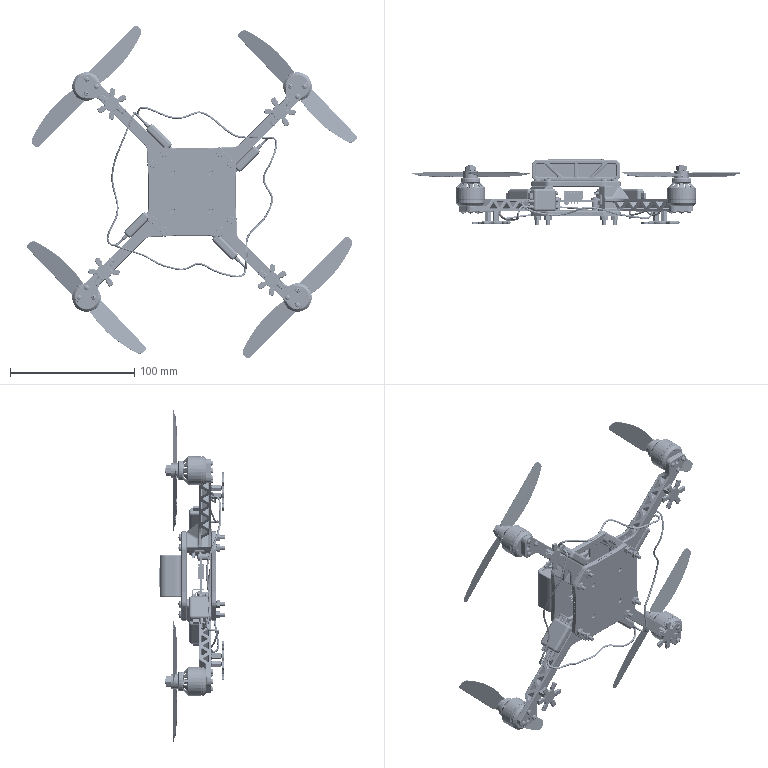Assembly | SolidWorks | mm | 79 component files | 87 solids | 8805 faces | box 265.01 x 53 x 267.04 mm | volume 145542 mm3 | plane 2963 | cylinder 2354 | torus 1852 | spline 1020 | cone 408 | sphere 208 | commonest cylinder face diameters 1 x1000 4 x200 2 x192 3 x136 0.2 x120 10 x82 2.2 x80 8 x48
Bill of materials:
1.Spider base | 1 |  | Thin flat plate with an octagon-like outline (chamfered corners, slightly concave long edges) and a pattern of through-holes: eight holes near the perimeter and four holes in an inner square pattern.
10.Motor | 4 |  | Cylindrical rotary-style body with a shaft running through it. One end has a chamfered, closed cap with circumferential grooves. The other end has an open spoked cage with a central boss. The flat end face has a ring of small holes around a central protruding shaft stub.
11.Distribution board | 2 |  | Thin square plate with rounded corners, a large through-hole at each corner, and a 3x6 grid of small holes near one edge. A small rectangular raised block on one face sits roughly above the hole grid region and has three small holes in its side face.
2.Spider top | 1 |  | Thin plate with an octagon-like outline that matches part-0's style (chamfered corners, slightly concave edges, eight perimeter holes). It has a large rounded-rectangle central cutout, two keyhole-like slotted cutouts above and below it, and a shallow recessed or raised inner octagonal step on one face.
3.Spider arm | 4 |  | Long tapered arm or bracket: a flat elongated plate with a row of triangular truss-style lightening pockets along a raised side web, a wider end pad with several holes, and a thicker block at the other end with a U-shaped channel or notch.
4.Battery | 1 |  | Rectangular block with rounded vertical edges. One face has four shallow pockets separated by diagonal and vertical ribs (a truss-like rib pattern). The other faces appear plain.
5.Spinner | 4 |  | Circular disc flange with a solid cylindrical shaft rising from the center of one face. The disc has four equally spaced through-holes on a circle, plus a small central hole or recess visible on the flange face.
6.Spacer | 4 |  | Plain cylindrical tube or sleeve with a concentric through-bore and flat, square-cut ends.
7.Electrical conector | 4 |  | Flat rounded-rectangular box-shaped body with cylindrical tube stubs coming out of two opposite edges (three on one side, two plus a rectangular tab or block on the other). Some stubs are visibly hollow.
8.Piller | 4 |  | Hexagonal standoff-like body with a cylindrical male stud with a chamfered tip at one end and a bored opening at the other end.
9.P | 4 |  | Two-blade propeller-like rotor: a central cylindrical hub with a through-bore and two thin, curved, tapered blades extending in opposite directions.
12.Electrical units | 1 |  | Pin-header-like part: a narrow plastic-style body made of five stacked segments with notched/chamfered profiles, and a straight square pin passing through each segment, extending on both sides (long on one side, shorter on the other).
13.Electrical unit 2 | 1 |  | Right-angle multi-row pin array: a rectangular block with 3 rows of 6 square-section pins. The pins pass straight through the block on one side and bend 90 degrees on the other, with each row bending at a different height so the rows nest.
Crijevo_paX | 1 |  | Long, thin, curved round-section strand with a short, slightly larger cylinder on each end. In some views it forms an S-shape or hook-shaped curves, and in one view it has a self-crossing loop.
Crijevo_paX2 | 1 |  | Long, thin, curved round-section strand with a short cylinder on each end. The path has wavy bends, hooked ends and, in one view, a tight fold.
Crijevo_paX3 | 1 |  | Long, thin, curved round-section strand with a short cylinder on each end. The path has several S-bends, end hooks and a loop where it crosses itself.
Crijevo_paX4 | 1 |  | Long, thin, curved round-section strand with a short cylinder on each end. The path has gentle waves, hooks at the ends and, in one view, a loop.
hex nut style 2_am_pkg | 8 |  | Hexagonal prism with a central through-bore and chamfered corners on both end faces; shaped like a hex nut.
hex nut style 2_am_pkg | 4 |  | Hexagonal prism with a central through-bore and chamfered corner edges; shaped like a hex nut and very similar to unnamed part 1.
pan cross head_am_pkg | 4 |  | Headed cylindrical pin: a plain round shank about four diameters long, with a larger round head that is short and has a domed top.
pan cross head_am_pkg | 8 |  | Long, slender headed pin: a plain round shank roughly ten or more diameters long, with a small domed round head at one end.
pan cross head_am_pkg | 12 |  | Domed (pan-style) round head with a cross-shaped recess, on a plain cylindrical shank about three diameters long; shaped like a cross-recess screw with no modeled thread.
pax_noga | 4 |  | Flat six-armed star-shaped plate with a central cylindrical pin standing up from one face. The arms are evenly spaced, have wavy side edges and flared ends, and all edges are rounded.
Mates:
1. concentric | 11.Distribution board-2 face at (15.25, 5.25, 15.25) dir (0, -1, 0) r 1.5 | 6.Spacer-4 face at (15.25, 11.25, 15.25) dir (0, -1, 0) r 2.5
2. concentric | 11.Distribution board-2 face at (15.25, 5.25, -15.25) dir (0, -1, 0) r 1.5 | 6.Spacer-1 face at (15.25, 11.25, -15.25) dir (0, -1, 0) r 2.5
3. concentric | 11.Distribution board-2 face at (15.25, 5.25, 15.25) dir (0, -1, 0) r 1.5 | 6.Spacer-4 face at (15.25, 11.25, 15.25) dir (0, -1, 0) r 2.5
4. coincident | 1.Spider base-2 face at (15.25, 3.5, 15.25) dir (0, 1, 0) | 11.Distribution board-2 face at (-16, 3.5, 16) dir (0, -1, 0)
5. concentric | 11.Distribution board-2 face at (15.25, 5.25, 15.25) dir (0, -1, 0) r 1.5 | Assembly 1-1/11.Distribution board-2 face at (15.25, 11.25, 15.25) dir (0, 1, 0) r 1.5
6. concentric | 11.Distribution board-2 face at (15.25, 5.25, -15.25) dir (0, -1, 0) r 1.5 | Assembly 1-1/11.Distribution board-2 face at (15.25, 11.25, -15.25) dir (0, 1, 0) r 1.5
7. concentric | 11.Distribution board-2 face at (15.25, 5.25, -15.25) dir (0, -1, 0) r 1.5 | 6.Spacer-1 face at (15.25, 11.25, -15.25) dir (0, -1, 0) r 1.5
8. coincident | 11.Distribution board-2 face at (-16, 5.25, 16) dir (0, 1, 0) | 6.Spacer-1 face at (15.25, 5.25, -15.25) dir (0, -1, 0)
9. coincident | Assembly 1-1/11.Distribution board-2 face at (16, 11.25, 16) dir (0, -1, 0) | 6.Spacer-1 face at (15.25, 11.25, -15.25) dir (0, 1, 0)
10. concentric | Assembly 1-1/11.Distribution board-2 face at (15.25, 11.25, -15.25) dir (0, 1, 0) r 1.5 | pan cross head_am_pkg-1 face at (15.25, 40.8, -15.25) dir (0, 1, 0) r 1.5
11. coincident | Assembly 1-1/11.Distribution board-2 face at (16, 13, 16) dir (0, 1, 0) | pan cross head_am_pkg-1 face at (13.817, 13, -14.806) dir (0, -1, 0)
12. concentric | 1.Spider base-2 face at (-22.627, 4, 31.113) dir (0, -1, 0) r 1.6 | 3.Spider arm-1 face at (-22.627, 14, 31.113) dir (0, -1, 0) r 1.5
13. concentric | 1.Spider base-2 face at (-31.113, 4, 22.627) dir (0, -1, 0) r 1.6 | 3.Spider arm-1 face at (-31.113, 14, 22.627) dir (0, -1, 0) r 1.5
14. coincident | 1.Spider base-2 face at (0, 4, 0) dir (0, 1, 0) | 3.Spider arm-1 face at (-46.062, 4, 31.92) dir (0, -1, 0)
15. concentric | 3.Spider arm-1 face at (-22.627, 14, 31.113) dir (0, -1, 0) r 1.5 | 2.Spider top-1 face at (-22.627, 24, 31.113) dir (0, 1, 0) r 1.6
16. concentric | 3.Spider arm-1 face at (-31.113, 14, 22.627) dir (0, -1, 0) r 1.5 | 2.Spider top-1 face at (-31.113, 24, 22.627) dir (0, 1, 0) r 1.6
17. coincident | 3.Spider arm-1 face at (-30.406, 24, 21.92) dir (0, 1, 0) | 2.Spider top-1 face at (0, 24, 0) dir (0, -1, 0)
18. concentric | 2.Spider top-1 face at (-22.627, 24, 31.113) dir (0, 1, 0) r 1.6 | pan cross head_am_pkg-8 face at (-22.627, 55.9, 31.113) dir (0, 1, 0) r 1.5
19. coincident | 2.Spider top-1 face at (0, 28.1, 0) dir (0, 1, 0) | pan cross head_am_pkg-8 face at (-21.417, 28.1, 30.227) dir (0, -1, 0)
20. concentric | 2.Spider top-1 face at (-22.627, 24, 31.113) dir (0, 1, 0) r 1.6 | hex nut style 2_am_pkg-1 face at (-22.627, 22.138, 31.113) dir (0, -1, 0) r 1.55
21. coincident | 1.Spider base-2 face at (0, 0, 0) dir (0, -1, 0) | hex nut style 2_am_pkg-1 face at (-25.776, 0, 31.521) dir (0, 1, 0)
22. concentric | 2.Spider top-1 face at (-31.113, 24, 22.627) dir (0, 1, 0) r 1.6 | pan cross head_am_pkg-12 face at (-31.113, 55.9, 22.627) dir (0, 1, 0) r 1.5
23. coincident | 2.Spider top-1 face at (0, 28.1, 0) dir (0, 1, 0) | pan cross head_am_pkg-12 face at (-30.091, 28.1, 21.53) dir (0, -1, 0)
24. concentric | pan cross head_am_pkg-12 face at (-31.113, 55.9, 22.627) dir (0, 1, 0) r 1.5 | hex nut style 2_am_pkg-12 face at (-31.113, 22.138, 22.627) dir (0, -1, 0) r 1.55
25. coincident | 1.Spider base-2 face at (0, 0, 0) dir (0, -1, 0) | hex nut style 2_am_pkg-12 face at (-34.128, 0, 23.622) dir (0, 1, 0)
26. concentric | 3.Spider arm-1 face at (-84.853, 14, 84.853) dir (0, -1, 0) r 2 | 10.Motor-1 face at (-84.853, 30.5, 84.853) dir (0, 1, 0) r 1
27. coincident | 3.Spider arm-1 face at (-83.291, 8.5, 70.563) dir (0, 1, 0) | 10.Motor-1 face at (-83.853, 8.5, 84.853) dir (0, -1, 0)
28. concentric | 3.Spider arm-1 face at (-76.853, 14, 84.853) dir (0, -1, 0) r 1.1 | 10.Motor-1 face at (-76.853, 11.5, 84.853) dir (0, -1, 0) r 1
29. concentric | 10.Motor-1 face at (-84.853, 11.5, 78.853) dir (0, -1, 0) r 1 | pan cross head_am_pkg-24 face at (-84.853, -23, 78.853) dir (0, -1, 0) r 1
30. coincident | 3.Spider arm-1 face at (-46.062, 4, 31.92) dir (0, -1, 0) | pan cross head_am_pkg-24 face at (-84.377, 4, 77.974) dir (0, 1, 0)
31. concentric | 3.Spider arm-1 face at (-84.853, 14, 90.853) dir (0, -1, 0) r 1.1 | pan cross head_am_pkg-28 face at (-84.853, -23, 90.853) dir (0, -1, 0) r 1
32. coincident | 3.Spider arm-1 face at (-46.062, 4, 31.92) dir (0, -1, 0) | pan cross head_am_pkg-28 face at (-84.085, 4, 91.493) dir (0, 1, 0)
33. concentric | 3.Spider arm-1 face at (-76.853, 14, 84.853) dir (0, -1, 0) r 1.1 | pan cross head_am_pkg-32 face at (-76.853, -23, 84.853) dir (0, -1, 0) r 1
34. coincident | 3.Spider arm-1 face at (-46.062, 4, 31.92) dir (0, -1, 0) | pan cross head_am_pkg-32 face at (-76.026, 4, 84.29) dir (0, 1, 0)
35. concentric | 10.Motor-1 face at (-84.853, 30.5, 84.853) dir (0, 1, 0) r 1 | 5.Spinner-1 face at (-84.853, 41.5, 84.853) dir (0, 1, 0) r 2
36. coincident | 10.Motor-1 face at (-77.353, 27, 84.853) dir (0, 1, 0) | 5.Spinner-1 face at (-84.853, 27, 84.853) dir (0, -1, 0)
37. concentric | 5.Spinner-1 face at (-84.853, 41.5, 84.853) dir (0, 1, 0) r 2 | 9.P-1 face at (-84.853, 36.5, 84.853) dir (0, -1, 0) r 2.5
38. coincident | 5.Spinner-1 face at (-76.853, 30.5, 84.898) dir (0, 1, 0) | 9.P-1 face at (-84.853, 30.5, 84.853) dir (0, -1, 0)
39. concentric | 5.Spinner-1 face at (-84.853, 41.5, 84.853) dir (0, 1, 0) r 2 | hex nut style 2_am_pkg-24 face at (-84.853, 15.462, 84.853) dir (0, 1, 0) r 2.05
40. concentric | 5.Spinner-1 face at (-84.853, 41.5, 84.853) dir (0, 1, 0) r 2 | hex nut style 2_am_pkg-24 face at (-84.853, 36.5, 84.853) dir (0, 1, 0) r 2
41. coincident | 9.P-1 face at (-84.853, 36.5, 84.853) dir (0, 1, 0) | hex nut style 2_am_pkg-24 face at (-85.114, 36.5, 88.886) dir (0, -1, 0)
42. coincident | 1.Spider base-2 plane at (0, 0, 0) dir (0, 0, 1) | assembly plane at (0, 0, 0) dir (0, 0, 1)
43. coincident | 1.Spider base-2 plane at (0, 0, 0) dir (1, 0, 0) | assembly plane at (0, 0, 0) dir (1, 0, 0)
44. coincident | 1.Spider base-2 plane at (0, 0, 0) dir (0, 1, 0) | assembly plane at (0, 0, 0) dir (0, 1, 0)
45. coincident | 3.Spider arm-1 face at (-81.625, 14, 94.353) dir (0.7071, 0, 0.7071) | 7.Electrical conector-1 face at (-21.92, 6, 34.648) dir (-0.7071, 0, -0.7071)
46. coincident | 3.Spider arm-1 face at (-46.062, 4, 31.92) dir (0, -1, 0) | 7.Electrical conector-1 face at (-36.062, 4, 48.79) dir (0, -1, 0)
47. coincident | 3.Spider arm-1 face at (-17.678, 14, 30.406) dir (0.7071, 0, -0.7071) | 7.Electrical conector-1 face at (-15.203, 7.5, 32.88) dir (0.7071, 0, -0.7071)
48. concentric | 3.Spider arm-1 face at (-64.407, 10, 70.771) dir (0, -1, 0) r 1.25 | 8.Piller-1 face at (-64.407, 4, 70.771) dir (0, 1, 0) r 1.25
49. coincident | 3.Spider arm-1 face at (-46.062, 4, 31.92) dir (0, -1, 0) | 8.Piller-1 face at (-64.407, 4, 70.771) dir (0, 1, 0)
50. concentric | 5.Spinner-2 face at (84.853, 41.5, 84.853) dir (0, 1, 0) r 2 | 9.P-4 face at (84.853, 36.5, 84.853) dir (0, -1, 0) r 2.5
51. coincident | 5.Spinner-2 face at (84.898, 30.5, 76.853) dir (0, 1, 0) | 9.P-4 face at (84.853, 30.5, 84.853) dir (0, -1, 0)
52. coincident | 2.Spider top-1 face at (0, 28.1, 0) dir (0, 1, 0) | 4.Battery-1 face at (0, 28.1, 0) dir (0, -1, 0)
53. width | 2.Spider top-1 face at (12.5, 24, -35) dir (0, 0, -1) | 2.Spider top-1 face at (-12.5, 24, 35) dir (0, 0, 1) | 4.Battery-1 face at (35.5, 45.6, -17) dir (0, 0, -1) | 4.Battery-1 face at (35.5, 45.6, 17) dir (0, 0, 1)
54. width | 2.Spider top-1 face at (-35, 24, -12.5) dir (-1, 0, 0) | 2.Spider top-1 face at (35, 24, 12.5) dir (1, 0, 0) | 4.Battery-1 face at (35.5, 45.6, -17) dir (1, 0, 0) | 4.Battery-1 face at (-35.5, 45.6, -17) dir (-1, 0, 0)
55. concentric | 8.Piller-2 face at (70.771, 0.8, 64.407) dir (0, -1, 0) r 1.25 | pax_noga-1 face at (70.771, -4.2, 64.407) dir (0, 1, 0) r 1.25
56. coincident | 8.Piller-2 face at (70.771, 0.8, 64.407) dir (0, -1, 0) | pax_noga-1 face at (70.771, 0.8, 64.407) dir (0, 1, 0)
57. concentric | Crijevo_paX-1 face at (-55.508, 11.9, -37.83) dir (0.7071, 0, 0.7071) r 1.1 | 7.Electrical conector-4 face at (-55.508, 11.9, -37.83) dir (0.7071, 0, 0.7071) r 1.1
58. coincident | 7.Electrical conector-4 face at (-50.205, 6, -37.477) dir (-0.7071, 0, -0.7071) | Crijevo_paX-1 face at (-52.679, 11.9, -35.002) dir (0.7071, 0, 0.7071)
59. parallel | 1.Spider base-2 face at (0, 4, 0) dir (0, 1, 0) | Crijevo_paX-1 plane at (-52.679, 11.9, -35.002) dir (0, 1, 0)
60. concentric | 7.Electrical conector-1 face at (-37.83, 11.9, 55.508) dir (0.7071, 0, -0.7071) r 1.1 | Crijevo_paX2-1 face at (-37.83, 11.9, 55.508) dir (0.7071, 0, -0.7071) r 1.1
61. coincident | 7.Electrical conector-1 face at (-37.477, 6, 50.205) dir (-0.7071, 0, 0.7071) | Crijevo_paX2-1 face at (-35.002, 11.9, 52.679) dir (0.7071, 0, -0.7071)
62. concentric | 7.Electrical conector-2 face at (55.508, 7.5, 37.83) dir (-0.7071, 0, -0.7071) r 1.1 | Crijevo_paX2-1 face at (52.679, 7.5, 35.002) dir (0.7071, 0, 0.7071) r 1.1
63. concentric | 7.Electrical conector-2 face at (55.508, 11.9, 37.83) dir (-0.7071, 0, -0.7071) r 1.1 | Crijevo_paX3-1 face at (55.508, 11.9, 37.83) dir (-0.7071, 0, -0.7071) r 1.1
64. concentric | 7.Electrical conector-3 face at (37.83, 7.5, -55.508) dir (-0.7071, 0, 0.7071) r 1.1 | Crijevo_paX3-1 face at (35.002, 7.5, -52.679) dir (0.7071, 0, -0.7071) r 1.1
65. concentric | 1.Spider base-2 face at (15.25, 0, 15.25) dir (0, 1, 0) r 1.5 | pan cross head_am_pkg-7 face at (15.25, 40.8, 15.25) dir (0, 1, 0) r 1.5
66. concentric | 7.Electrical conector-4 face at (-55.508, 7.5, -37.83) dir (0.7071, 0, 0.7071) r 1.1 | Crijevo_paX4-1 face at (-52.679, 7.5, -35.002) dir (-0.7071, 0, -0.7071) r 1.1
67. concentric | 7.Electrical conector-3 face at (37.83, 11.9, -55.508) dir (-0.7071, 0, 0.7071) r 1.5 | Crijevo_paX4-1 face at (37.83, 11.9, -55.508) dir (-0.7071, 0, 0.7071) r 1.1
68. width | 11.Distribution board-2 face at (0.7186, -12.176, 66.144) dir (-0.1122, 0.8582, -0.5008) | 11.Distribution board-2 face at (0.9149, -13.678, 67.021) dir (0.1122, -0.8582, 0.5008) | 12.Electrical units-2 face at (38.13, 2.657, 83.044) dir (0.1122, -0.8582, 0.5008) | 12.Electrical units-2 face at (38.342, 1.034, 83.99) dir (-0.1122, 0.8582, -0.5008)
69. coincident | 11.Distribution board-2 face at (32.563, -4.594, 75.499) dir (0.9308, 0.2672, 0.2494) | 12.Electrical units-2 face at (26.545, 2.705, 90.144) dir (-0.9308, -0.2672, -0.2494)
70. distance | 12.Electrical units-2 face at (32.476, 1.205, 79.635) dir (0.3478, -0.4382, -0.8288) | 11.Distribution board-2 face at (1.611, -14.554, 65.363) dir (0.3478, -0.4382, -0.8288)
71. parallel | 11.Distribution board-2 face at (-0.9468, -14.212, 66.522) dir (-0.9308, -0.2672, -0.2494) | 13.Electrical unit 2-2 face at (-2.881, 13.065, 95.688) dir (-0.9308, -0.2672, -0.2494)
72. parallel | 11.Distribution board-2 face at (-10.911, 1.222, 95.202) dir (-0.3478, 0.4382, 0.8288) | 13.Electrical unit 2-2 face at (-0.5572, 4.671, 101.101) dir (-0.3478, 0.4382, 0.8288)
73. distance | 13.Electrical unit 2-2 face at (0.3124, 3.576, 99.028) dir (0.3478, -0.4382, -0.8288) | 11.Distribution board-2 face at (-10.911, 1.222, 95.202) dir (-0.3478, 0.4382, 0.8288)
74. distance | 13.Electrical unit 2-2 face at (11.305, 17.136, 99.488) dir (0.9308, 0.2672, 0.2494) | 11.Distribution board-2 face at (32.563, -4.594, 75.499) dir (0.9308, 0.2672, 0.2494)
75. distance | 11.Distribution board-2 face at (0.9149, -13.678, 67.021) dir (0.1122, -0.8582, 0.5008) | 13.Electrical unit 2-2 face at (-1.617, 7.087, 99.379) dir (0.1122, -0.8582, 0.5008)